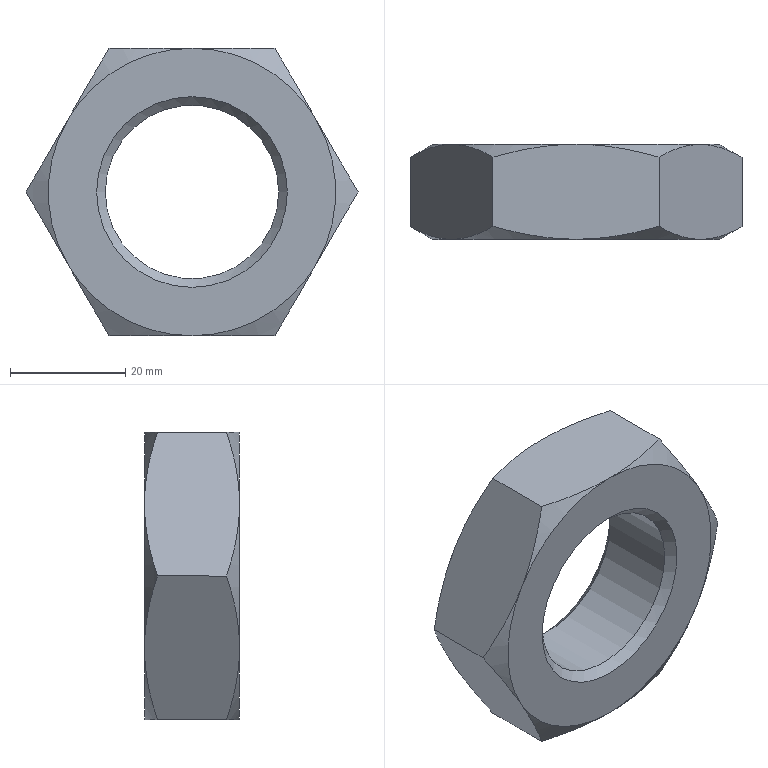Component | NX | GB-T6172_1-2000_M33X3_5_2 | 1 solid | 23 faces | volume 23438 mm3 | cone 14 | plane 8 | cylinder 1 | commonest cylinder face diameters 30.158 x1